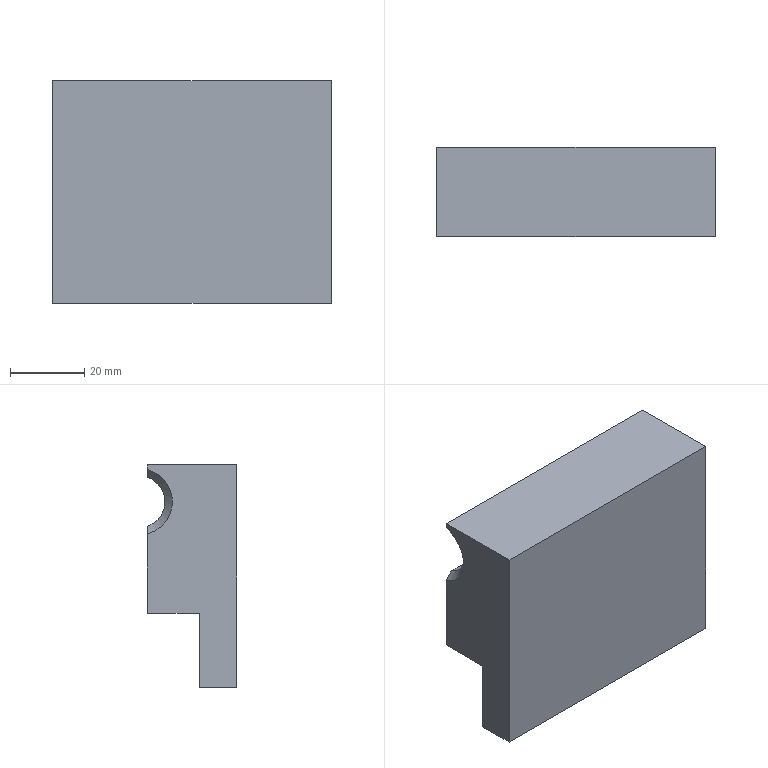Component | SolidWorks | HZ022-HFP20-1_HZ022-A001-E008-1 | 1 solid | 12 faces | box 75 x 24 x 60 mm | volume 83536 mm3 | plane 9 | cone 2 | cylinder 1 | commonest cylinder face diameters 13.9 x1 | material AL6061
build123d program:
from build123d import *

# Parameters (mm, degrees)
SKETCH1_W           = 75
SKETCH1_H           = 60
BOSS_EXTRUDE1_DEPTH = 10
SKETCH2_W           = 75
SKETCH2_H           = 40
BOSS_EXTRUDE2_DEPTH = 14
SKETCH3_R           = 6.95
CUT_EXTRUDE1_DEPTH  = 82.982
CHAMFER1_SIZE       = 2


with BuildPart() as part:
    # Sketch1 → Boss-Extrude1 (new body)
    with BuildSketch(Plane(origin=(0, 0, 0), x_dir=(1, 0, 0), z_dir=(0, 1, 0))):
        Rectangle(SKETCH1_W, SKETCH1_H)
    extrude(amount=BOSS_EXTRUDE1_DEPTH)

    # Sketch2 → Boss-Extrude2 (add)
    with BuildSketch(Plane.XZ):
        with Locations((0, 10)):
            Rectangle(SKETCH2_W, SKETCH2_H)
    extrude(amount=BOSS_EXTRUDE2_DEPTH)

    # Sketch3 → Cut-Extrude1 (cut, through all)
    with BuildSketch(Plane(origin=(37.5, 0, 0), x_dir=(0, 0, -1), z_dir=(1, 0, 0))):
        with Locations((-20, -16.25)):
            Circle(SKETCH3_R)
    extrude(amount=-CUT_EXTRUDE1_DEPTH, mode=Mode.SUBTRACT)

    # Chamfer1
    chamfer1_edges = [part.edges().sort_by_distance(p)[0] for p in [
        (-37.5, -9.3, 20),
        (37.5, -9.3, 20),
    ]]
    chamfer(chamfer1_edges, length=CHAMFER1_SIZE)


solid = part.part

# Placed as in the assembly
solid = solid.moved(Location((117.944, 110.402, 907), (0, 0, 180)))
STEP:
#1=CARTESIAN_POINT('',(6.041,4.898,36.237));
#2=VERTEX_POINT('',#1);
#3=CARTESIAN_POINT('',(3.246,4.898,36.237));
#4=VERTEX_POINT('',#3);
#5=CARTESIAN_POINT('',(6.12,4.898,36.237));
#6=DIRECTION('',(-1.,-0.,0.));
#7=VECTOR('',#6,39.37);
#8=LINE('',#5,#7);
#9=EDGE_CURVE('',#2,#4,#8,.T.);
#10=ORIENTED_EDGE('',*,*,#9,.F.);
#11=CARTESIAN_POINT('',(6.12,4.898,36.155));
#12=VERTEX_POINT('',#11);
#13=CARTESIAN_POINT('',(6.041,4.898,36.237));
#14=CARTESIAN_POINT('',(6.067,4.898,36.21));
#15=CARTESIAN_POINT('',(6.093,4.898,36.182));
#16=CARTESIAN_POINT('',(6.12,4.898,36.155));
#17=B_SPLINE_CURVE_WITH_KNOTS('',3,(#13,#14,#15,#16),.UNSPECIFIED.,.F.,.F.,(4,4),(0.,0.00289),.UNSPECIFIED.);
#18=EDGE_CURVE('',#2,#12,#17,.T.);
#19=ORIENTED_EDGE('',*,*,#18,.T.);
#20=CARTESIAN_POINT('',(6.12,4.898,35.315));
#21=VERTEX_POINT('',#20);
#22=CARTESIAN_POINT('',(6.12,4.898,36.89));
#23=DIRECTION('',(-0.,0.,-1.));
#24=VECTOR('',#23,39.37);
#25=LINE('',#22,#24);
#26=EDGE_CURVE('',#12,#21,#25,.T.);
#27=ORIENTED_EDGE('',*,*,#26,.T.);
#28=CARTESIAN_POINT('',(3.167,4.898,35.315));
#29=VERTEX_POINT('',#28);
#30=CARTESIAN_POINT('',(6.12,4.898,35.315));
#31=DIRECTION('',(-1.,-0.,0.));
#32=VECTOR('',#31,39.37);
#33=LINE('',#30,#32);
#34=EDGE_CURVE('',#21,#29,#33,.T.);
#35=ORIENTED_EDGE('',*,*,#34,.T.);
#36=CARTESIAN_POINT('',(3.167,4.898,36.155));
#37=VERTEX_POINT('',#36);
#38=CARTESIAN_POINT('',(3.167,4.898,36.89));
#39=DIRECTION('',(0.,-0.,1.));
#40=VECTOR('',#39,39.37);
#41=LINE('',#38,#40);
#42=EDGE_CURVE('',#29,#37,#41,.T.);
#43=ORIENTED_EDGE('',*,*,#42,.T.);
#44=CARTESIAN_POINT('',(3.167,4.898,36.155));
#45=CARTESIAN_POINT('',(3.193,4.898,36.182));
#46=CARTESIAN_POINT('',(3.22,4.898,36.21));
#47=CARTESIAN_POINT('',(3.246,4.898,36.237));
#48=B_SPLINE_CURVE_WITH_KNOTS('',3,(#44,#45,#46,#47),.UNSPECIFIED.,.F.,.F.,(4,4),(0.,0.00289),.UNSPECIFIED.);
#49=EDGE_CURVE('',#37,#4,#48,.T.);
#50=ORIENTED_EDGE('',*,*,#49,.T.);
#51=EDGE_LOOP('',(#10,#19,#27,#35,#43,#50));
#52=FACE_OUTER_BOUND('',#51,.T.);
#53=CARTESIAN_POINT('',(4.643,4.898,35.709));
#54=DIRECTION('',(-0.,1.,0.));
#55=DIRECTION('',(-0.,0.,-1.));
#56=AXIS2_PLACEMENT_3D('',#53,#54,#55);
#57=PLANE('',#56);
#58=ADVANCED_FACE('',(#52),#57,.T.);
#59=CARTESIAN_POINT('',(6.12,4.347,35.315));
#60=VERTEX_POINT('',#59);
#61=CARTESIAN_POINT('',(3.167,4.347,35.315));
#62=VERTEX_POINT('',#61);
#63=CARTESIAN_POINT('',(6.12,4.347,35.315));
#64=DIRECTION('',(-1.,-0.,0.));
#65=VECTOR('',#64,39.37);
#66=LINE('',#63,#65);
#67=EDGE_CURVE('',#60,#62,#66,.T.);
#68=ORIENTED_EDGE('',*,*,#67,.F.);
#69=CARTESIAN_POINT('',(6.12,4.347,34.528));
#70=VERTEX_POINT('',#69);
#71=CARTESIAN_POINT('',(6.12,4.347,34.528));
#72=DIRECTION('',(0.,-0.,1.));
#73=VECTOR('',#72,39.37);
#74=LINE('',#71,#73);
#75=EDGE_CURVE('',#70,#60,#74,.T.);
#76=ORIENTED_EDGE('',*,*,#75,.F.);
#77=CARTESIAN_POINT('',(3.167,4.347,34.528));
#78=VERTEX_POINT('',#77);
#79=CARTESIAN_POINT('',(6.12,4.347,34.528));
#80=DIRECTION('',(1.,0.,-0.));
#81=VECTOR('',#80,39.37);
#82=LINE('',#79,#81);
#83=EDGE_CURVE('',#78,#70,#82,.T.);
#84=ORIENTED_EDGE('',*,*,#83,.F.);
#85=CARTESIAN_POINT('',(3.167,4.347,34.528));
#86=DIRECTION('',(-0.,0.,-1.));
#87=VECTOR('',#86,39.37);
#88=LINE('',#85,#87);
#89=EDGE_CURVE('',#62,#78,#88,.T.);
#90=ORIENTED_EDGE('',*,*,#89,.F.);
#91=EDGE_LOOP('',(#68,#76,#84,#90));
#92=FACE_OUTER_BOUND('',#91,.T.);
#93=CARTESIAN_POINT('',(4.643,4.347,35.709));
#94=DIRECTION('',(0.,-1.,-0.));
#95=DIRECTION('',(0.,-0.,1.));
#96=AXIS2_PLACEMENT_3D('',#93,#94,#95);
#97=PLANE('',#96);
#98=ADVANCED_FACE('',(#92),#97,.F.);
#99=CARTESIAN_POINT('',(3.167,4.898,36.837));
#100=VERTEX_POINT('',#99);
#101=CARTESIAN_POINT('',(3.167,4.898,36.89));
#102=VERTEX_POINT('',#101);
#103=CARTESIAN_POINT('',(3.167,4.898,36.89));
#104=DIRECTION('',(0.,-0.,1.));
#105=VECTOR('',#104,39.37);
#106=LINE('',#103,#105);
#107=EDGE_CURVE('',#100,#102,#106,.T.);
#108=ORIENTED_EDGE('',*,*,#107,.F.);
#109=CARTESIAN_POINT('',(3.167,4.986,36.496));
#110=DIRECTION('',(1.,0.,-0.));
#111=DIRECTION('',(0.,0.,1.));
#112=AXIS2_PLACEMENT_3D('',#109,#110,#111);
#113=CIRCLE('',#112,0.3524);
#114=EDGE_CURVE('',#100,#37,#113,.T.);
#115=ORIENTED_EDGE('',*,*,#114,.T.);
#116=ORIENTED_EDGE('',*,*,#42,.F.);
#117=CARTESIAN_POINT('',(3.167,4.898,35.315));
#118=DIRECTION('',(0.,-1.,-0.));
#119=VECTOR('',#118,39.37);
#120=LINE('',#117,#119);
#121=EDGE_CURVE('',#29,#62,#120,.T.);
#122=ORIENTED_EDGE('',*,*,#121,.T.);
#123=ORIENTED_EDGE('',*,*,#89,.T.);
#124=CARTESIAN_POINT('',(3.167,3.953,34.528));
#125=VERTEX_POINT('',#124);
#126=CARTESIAN_POINT('',(3.167,3.953,34.528));
#127=DIRECTION('',(-0.,1.,0.));
#128=VECTOR('',#127,39.37);
#129=LINE('',#126,#128);
#130=EDGE_CURVE('',#125,#78,#129,.T.);
#131=ORIENTED_EDGE('',*,*,#130,.F.);
#132=CARTESIAN_POINT('',(3.167,3.953,36.89));
#133=VERTEX_POINT('',#132);
#134=CARTESIAN_POINT('',(3.167,3.953,34.528));
#135=DIRECTION('',(-0.,0.,-1.));
#136=VECTOR('',#135,39.37);
#137=LINE('',#134,#136);
#138=EDGE_CURVE('',#133,#125,#137,.T.);
#139=ORIENTED_EDGE('',*,*,#138,.F.);
#140=CARTESIAN_POINT('',(3.167,3.953,36.89));
#141=DIRECTION('',(-0.,1.,0.));
#142=VECTOR('',#141,39.37);
#143=LINE('',#140,#142);
#144=EDGE_CURVE('',#133,#102,#143,.T.);
#145=ORIENTED_EDGE('',*,*,#144,.T.);
#146=EDGE_LOOP('',(#108,#115,#116,#122,#123,#131,#139,#145));
#147=FACE_OUTER_BOUND('',#146,.T.);
#148=CARTESIAN_POINT('',(3.167,3.953,34.528));
#149=DIRECTION('',(1.,0.,-0.));
#150=DIRECTION('',(0.,-0.,1.));
#151=AXIS2_PLACEMENT_3D('',#148,#149,#150);
#152=PLANE('',#151);
#153=ADVANCED_FACE('',(#147),#152,.F.);
#154=ORIENTED_EDGE('',*,*,#83,.T.);
#155=CARTESIAN_POINT('',(6.12,3.953,34.528));
#156=VERTEX_POINT('',#155);
#157=CARTESIAN_POINT('',(6.12,3.953,34.528));
#158=DIRECTION('',(-0.,1.,0.));
#159=VECTOR('',#158,39.37);
#160=LINE('',#157,#159);
#161=EDGE_CURVE('',#156,#70,#160,.T.);
#162=ORIENTED_EDGE('',*,*,#161,.F.);
#163=CARTESIAN_POINT('',(6.12,3.953,34.528));
#164=DIRECTION('',(1.,0.,-0.));
#165=VECTOR('',#164,39.37);
#166=LINE('',#163,#165);
#167=EDGE_CURVE('',#125,#156,#166,.T.);
#168=ORIENTED_EDGE('',*,*,#167,.F.);
#169=ORIENTED_EDGE('',*,*,#130,.T.);
#170=EDGE_LOOP('',(#154,#162,#168,#169));
#171=FACE_OUTER_BOUND('',#170,.T.);
#172=CARTESIAN_POINT('',(6.12,3.953,34.528));
#173=DIRECTION('',(0.,-0.,1.));
#174=DIRECTION('',(-1.,-0.,0.));
#175=AXIS2_PLACEMENT_3D('',#172,#173,#174);
#176=PLANE('',#175);
#177=ADVANCED_FACE('',(#171),#176,.F.);
#178=ORIENTED_EDGE('',*,*,#26,.F.);
#179=CARTESIAN_POINT('',(6.12,4.898,36.837));
#180=VERTEX_POINT('',#179);
#181=CARTESIAN_POINT('',(6.12,4.986,36.496));
#182=DIRECTION('',(-1.,-0.,0.));
#183=DIRECTION('',(-0.,0.,-1.));
#184=AXIS2_PLACEMENT_3D('',#181,#182,#183);
#185=CIRCLE('',#184,0.3524);
#186=EDGE_CURVE('',#12,#180,#185,.T.);
#187=ORIENTED_EDGE('',*,*,#186,.T.);
#188=CARTESIAN_POINT('',(6.12,4.898,36.89));
#189=VERTEX_POINT('',#188);
#190=CARTESIAN_POINT('',(6.12,4.898,36.89));
#191=DIRECTION('',(-0.,0.,-1.));
#192=VECTOR('',#191,39.37);
#193=LINE('',#190,#192);
#194=EDGE_CURVE('',#189,#180,#193,.T.);
#195=ORIENTED_EDGE('',*,*,#194,.F.);
#196=CARTESIAN_POINT('',(6.12,3.953,36.89));
#197=VERTEX_POINT('',#196);
#198=CARTESIAN_POINT('',(6.12,3.953,36.89));
#199=DIRECTION('',(-0.,1.,0.));
#200=VECTOR('',#199,39.37);
#201=LINE('',#198,#200);
#202=EDGE_CURVE('',#197,#189,#201,.T.);
#203=ORIENTED_EDGE('',*,*,#202,.F.);
#204=CARTESIAN_POINT('',(6.12,3.953,34.528));
#205=DIRECTION('',(0.,-0.,1.));
#206=VECTOR('',#205,39.37);
#207=LINE('',#204,#206);
#208=EDGE_CURVE('',#156,#197,#207,.T.);
#209=ORIENTED_EDGE('',*,*,#208,.F.);
#210=ORIENTED_EDGE('',*,*,#161,.T.);
#211=ORIENTED_EDGE('',*,*,#75,.T.);
#212=CARTESIAN_POINT('',(6.12,4.898,35.315));
#213=DIRECTION('',(0.,-1.,-0.));
#214=VECTOR('',#213,39.37);
#215=LINE('',#212,#214);
#216=EDGE_CURVE('',#21,#60,#215,.T.);
#217=ORIENTED_EDGE('',*,*,#216,.F.);
#218=EDGE_LOOP('',(#178,#187,#195,#203,#209,#210,#211,#217));
#219=FACE_OUTER_BOUND('',#218,.T.);
#220=CARTESIAN_POINT('',(6.12,3.953,34.528));
#221=DIRECTION('',(-1.,-0.,0.));
#222=DIRECTION('',(-0.,0.,-1.));
#223=AXIS2_PLACEMENT_3D('',#220,#221,#222);
#224=PLANE('',#223);
#225=ADVANCED_FACE('',(#219),#224,.F.);
#226=ORIENTED_EDGE('',*,*,#202,.T.);
#227=CARTESIAN_POINT('',(6.12,4.898,36.89));
#228=DIRECTION('',(1.,0.,-0.));
#229=VECTOR('',#228,39.37);
#230=LINE('',#227,#229);
#231=EDGE_CURVE('',#102,#189,#230,.T.);
#232=ORIENTED_EDGE('',*,*,#231,.F.);
#233=ORIENTED_EDGE('',*,*,#144,.F.);
#234=CARTESIAN_POINT('',(6.12,3.953,36.89));
#235=DIRECTION('',(-1.,-0.,0.));
#236=VECTOR('',#235,39.37);
#237=LINE('',#234,#236);
#238=EDGE_CURVE('',#197,#133,#237,.T.);
#239=ORIENTED_EDGE('',*,*,#238,.F.);
#240=EDGE_LOOP('',(#226,#232,#233,#239));
#241=FACE_OUTER_BOUND('',#240,.T.);
#242=CARTESIAN_POINT('',(6.12,3.953,36.89));
#243=DIRECTION('',(-0.,0.,-1.));
#244=DIRECTION('',(1.,0.,-0.));
#245=AXIS2_PLACEMENT_3D('',#242,#243,#244);
#246=PLANE('',#245);
#247=ADVANCED_FACE('',(#241),#246,.F.);
#248=ORIENTED_EDGE('',*,*,#138,.T.);
#249=ORIENTED_EDGE('',*,*,#167,.T.);
#250=ORIENTED_EDGE('',*,*,#208,.T.);
#251=ORIENTED_EDGE('',*,*,#238,.T.);
#252=EDGE_LOOP('',(#248,#249,#250,#251));
#253=FACE_OUTER_BOUND('',#252,.T.);
#254=CARTESIAN_POINT('',(4.643,3.953,35.709));
#255=DIRECTION('',(0.,-1.,-0.));
#256=DIRECTION('',(0.,-0.,1.));
#257=AXIS2_PLACEMENT_3D('',#254,#255,#256);
#258=PLANE('',#257);
#259=ADVANCED_FACE('',(#253),#258,.T.);
#260=ORIENTED_EDGE('',*,*,#67,.T.);
#261=ORIENTED_EDGE('',*,*,#121,.F.);
#262=ORIENTED_EDGE('',*,*,#34,.F.);
#263=ORIENTED_EDGE('',*,*,#216,.T.);
#264=EDGE_LOOP('',(#260,#261,#262,#263));
#265=FACE_OUTER_BOUND('',#264,.T.);
#266=CARTESIAN_POINT('',(6.12,4.898,35.315));
#267=DIRECTION('',(0.,-0.,1.));
#268=DIRECTION('',(-1.,-0.,0.));
#269=AXIS2_PLACEMENT_3D('',#266,#267,#268);
#270=PLANE('',#269);
#271=ADVANCED_FACE('',(#265),#270,.F.);
#272=ORIENTED_EDGE('',*,*,#194,.T.);
#273=CARTESIAN_POINT('',(6.041,4.898,36.755));
#274=VERTEX_POINT('',#273);
#275=CARTESIAN_POINT('',(6.12,4.898,36.837));
#276=CARTESIAN_POINT('',(6.093,4.898,36.81));
#277=CARTESIAN_POINT('',(6.067,4.898,36.783));
#278=CARTESIAN_POINT('',(6.041,4.898,36.755));
#279=B_SPLINE_CURVE_WITH_KNOTS('',3,(#275,#276,#277,#278),.UNSPECIFIED.,.F.,.F.,(4,4),(0.,0.00289),.UNSPECIFIED.);
#280=EDGE_CURVE('',#180,#274,#279,.T.);
#281=ORIENTED_EDGE('',*,*,#280,.T.);
#282=CARTESIAN_POINT('',(3.246,4.898,36.755));
#283=VERTEX_POINT('',#282);
#284=CARTESIAN_POINT('',(6.12,4.898,36.755));
#285=DIRECTION('',(1.,0.,-0.));
#286=VECTOR('',#285,39.37);
#287=LINE('',#284,#286);
#288=EDGE_CURVE('',#283,#274,#287,.T.);
#289=ORIENTED_EDGE('',*,*,#288,.F.);
#290=CARTESIAN_POINT('',(3.246,4.898,36.755));
#291=CARTESIAN_POINT('',(3.22,4.898,36.783));
#292=CARTESIAN_POINT('',(3.193,4.898,36.81));
#293=CARTESIAN_POINT('',(3.167,4.898,36.837));
#294=B_SPLINE_CURVE_WITH_KNOTS('',3,(#290,#291,#292,#293),.UNSPECIFIED.,.F.,.F.,(4,4),(0.,0.00289),.UNSPECIFIED.);
#295=EDGE_CURVE('',#283,#100,#294,.T.);
#296=ORIENTED_EDGE('',*,*,#295,.T.);
#297=ORIENTED_EDGE('',*,*,#107,.T.);
#298=ORIENTED_EDGE('',*,*,#231,.T.);
#299=EDGE_LOOP('',(#272,#281,#289,#296,#297,#298));
#300=FACE_OUTER_BOUND('',#299,.T.);
#301=CARTESIAN_POINT('',(4.643,4.898,35.709));
#302=DIRECTION('',(-0.,1.,0.));
#303=DIRECTION('',(-0.,0.,-1.));
#304=AXIS2_PLACEMENT_3D('',#301,#302,#303);
#305=PLANE('',#304);
#306=ADVANCED_FACE('',(#300),#305,.T.);
#307=ORIENTED_EDGE('',*,*,#288,.T.);
#308=CARTESIAN_POINT('',(6.041,4.986,36.496));
#309=DIRECTION('',(1.,0.,-0.));
#310=DIRECTION('',(-0.,-0.,-1.));
#311=AXIS2_PLACEMENT_3D('',#308,#309,#310);
#312=CIRCLE('',#311,0.2736);
#313=EDGE_CURVE('',#274,#2,#312,.T.);
#314=ORIENTED_EDGE('',*,*,#313,.T.);
#315=ORIENTED_EDGE('',*,*,#9,.T.);
#316=CARTESIAN_POINT('',(3.246,4.986,36.496));
#317=DIRECTION('',(-1.,-0.,0.));
#318=DIRECTION('',(0.,-0.,1.));
#319=AXIS2_PLACEMENT_3D('',#316,#317,#318);
#320=CIRCLE('',#319,0.2736);
#321=EDGE_CURVE('',#4,#283,#320,.T.);
#322=ORIENTED_EDGE('',*,*,#321,.T.);
#323=EDGE_LOOP('',(#307,#314,#315,#322));
#324=FACE_OUTER_BOUND('',#323,.T.);
#325=CARTESIAN_POINT('',(6.12,4.986,36.496));
#326=DIRECTION('',(-1.,-0.,0.));
#327=DIRECTION('',(-0.,0.,-1.));
#328=AXIS2_PLACEMENT_3D('',#325,#326,#327);
#329=CYLINDRICAL_SURFACE('',#328,0.2736);
#330=ADVANCED_FACE('',(#324),#329,.F.);
#331=ORIENTED_EDGE('',*,*,#18,.F.);
#332=ORIENTED_EDGE('',*,*,#313,.F.);
#333=ORIENTED_EDGE('',*,*,#280,.F.);
#334=ORIENTED_EDGE('',*,*,#186,.F.);
#335=EDGE_LOOP('',(#331,#332,#333,#334));
#336=FACE_OUTER_BOUND('',#335,.T.);
#337=CARTESIAN_POINT('',(6.12,4.986,36.496));
#338=DIRECTION('',(1.,0.,-0.));
#339=DIRECTION('',(0.,0.,1.));
#340=AXIS2_PLACEMENT_3D('',#337,#338,#339);
#341=CONICAL_SURFACE('',#340,0.3524,0.7854);
#342=ADVANCED_FACE('',(#336),#341,.F.);
#343=ORIENTED_EDGE('',*,*,#49,.F.);
#344=ORIENTED_EDGE('',*,*,#114,.F.);
#345=ORIENTED_EDGE('',*,*,#295,.F.);
#346=ORIENTED_EDGE('',*,*,#321,.F.);
#347=EDGE_LOOP('',(#343,#344,#345,#346));
#348=FACE_OUTER_BOUND('',#347,.T.);
#349=CARTESIAN_POINT('',(3.246,4.986,36.496));
#350=DIRECTION('',(-1.,-0.,0.));
#351=DIRECTION('',(-0.,0.,-1.));
#352=AXIS2_PLACEMENT_3D('',#349,#350,#351);
#353=CONICAL_SURFACE('',#352,0.2736,0.7854);
#354=ADVANCED_FACE('',(#348),#353,.F.);
#355=CLOSED_SHELL('',(#58,#98,#153,#177,#225,#247,#259,#271,#306,#330,#342,#354));
#356=MANIFOLD_SOLID_BREP('',#355);
#357=CARTESIAN_POINT('',(0.,0.,0.));
#358=DIRECTION('',(0.,0.,1.));
#359=DIRECTION('',(1.,0.,0.));
#360=AXIS2_PLACEMENT_3D('',#357,#358,#359);
#361=(LENGTH_UNIT()NAMED_UNIT(*)SI_UNIT($,.METRE.));
#362=LENGTH_MEASURE_WITH_UNIT(LENGTH_MEASURE(0.0254),#361);
#363=DIMENSIONAL_EXPONENTS(1.,0.,0.,0.,0.,0.,0.);
#364=(CONVERSION_BASED_UNIT('',#362)LENGTH_UNIT()NAMED_UNIT(#363));
#365=UNCERTAINTY_MEASURE_WITH_UNIT(LENGTH_MEASURE(0.00001),#364,'','');
#366=(NAMED_UNIT(*)PLANE_ANGLE_UNIT()SI_UNIT($,.RADIAN.));
#367=(NAMED_UNIT(*)SI_UNIT($,.STERADIAN.)SOLID_ANGLE_UNIT());
#368=(GEOMETRIC_REPRESENTATION_CONTEXT(3)GLOBAL_UNCERTAINTY_ASSIGNED_CONTEXT((#365))GLOBAL_UNIT_ASSIGNED_CONTEXT((#364,#366,#367))REPRESENTATION_CONTEXT('',''));
#369=ADVANCED_BREP_SHAPE_REPRESENTATION('',(#356,#360),#368);
#370=COLOUR_RGB('',0.7922,0.8196,0.9333);
#371=FILL_AREA_STYLE_COLOUR('',#370);
#372=FILL_AREA_STYLE('',(#371));
#373=SURFACE_STYLE_FILL_AREA(#372);
#374=SURFACE_SIDE_STYLE('',(#373));
#375=SURFACE_STYLE_USAGE(.BOTH.,#374);
#376=PRESENTATION_STYLE_ASSIGNMENT((#375));
#377=STYLED_ITEM('',(#376),#356);
#378=(LENGTH_UNIT()NAMED_UNIT(*)SI_UNIT($,.METRE.));
#379=LENGTH_MEASURE_WITH_UNIT(LENGTH_MEASURE(0.0254),#378);
#380=DIMENSIONAL_EXPONENTS(1.,0.,0.,0.,0.,0.,0.);
#381=(CONVERSION_BASED_UNIT('',#379)LENGTH_UNIT()NAMED_UNIT(#380));
#382=UNCERTAINTY_MEASURE_WITH_UNIT(LENGTH_MEASURE(0.00001),#381,'','');
#383=(NAMED_UNIT(*)PLANE_ANGLE_UNIT()SI_UNIT($,.RADIAN.));
#384=(NAMED_UNIT(*)SI_UNIT($,.STERADIAN.)SOLID_ANGLE_UNIT());
#385=(GEOMETRIC_REPRESENTATION_CONTEXT(3)GLOBAL_UNCERTAINTY_ASSIGNED_CONTEXT((#382))GLOBAL_UNIT_ASSIGNED_CONTEXT((#381,#383,#384))REPRESENTATION_CONTEXT('',''));
#386=MECHANICAL_DESIGN_GEOMETRIC_PRESENTATION_REPRESENTATION('',(#377),#385);
#387=PRESENTATION_LAYER_ASSIGNMENT('','',(#377));